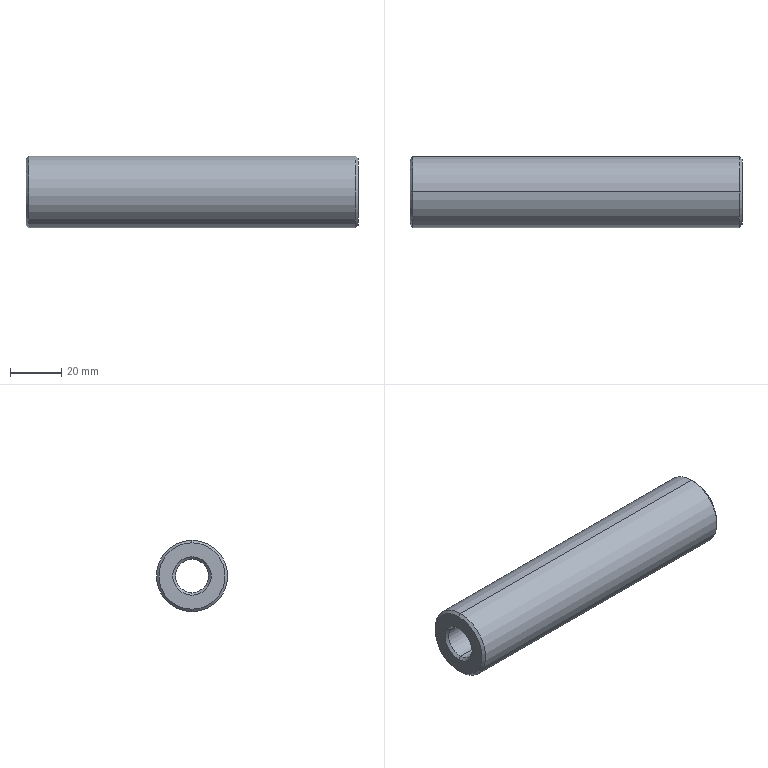Component | SolidWorks | LocatingGuideBushing130-2 | 1 solid | 14 faces | box 130 x 28 x 28 mm | volume 62664 mm3 | cone 8 | cylinder 4 | plane 2 | commonest cylinder face diameters 13 x2 28 x2
build123d program:
from build123d import *

# Parameters (mm, degrees)
SKETCH1_R           = 14
SKETCH1_R_2         = 6.5
BOSS_EXTRUDE1_DEPTH = 130
CHAMFER1_SIZE       = 1


with BuildPart() as part:
    # Sketch1 → Boss-Extrude1 (new body)
    with BuildSketch(Plane.XY):
        Circle(SKETCH1_R)
        Circle(SKETCH1_R_2, mode=Mode.SUBTRACT)
    extrude(amount=BOSS_EXTRUDE1_DEPTH)

    # Chamfer1
    chamfer1_edges = [part.edges().sort_by_distance(p)[0] for p in [
        (-14, 0, 0),
        (-14, 0, 130),
        (-6.5, 0, 0),
        (-6.5, 0, 130),
    ]]
    chamfer(chamfer1_edges, length=CHAMFER1_SIZE)


solid = part.part

# Placed as in the assembly
solid = solid.moved(Location((-197.809, 220.819, 0), (0, 90, 0)))
STEP:
#1=CARTESIAN_POINT('',(-2.67,8.694,-0.5118));
#2=VERTEX_POINT('',#1);
#3=CARTESIAN_POINT('',(-2.67,8.694,0.5118));
#4=VERTEX_POINT('',#3);
#5=CARTESIAN_POINT('',(-2.67,8.694,0.));
#6=DIRECTION('',(1.,-0.,0.));
#7=DIRECTION('',(0.,0.,-1.));
#8=AXIS2_PLACEMENT_3D('',#5,#6,#7);
#9=CIRCLE('',#8,0.5118);
#10=EDGE_CURVE('',#2,#4,#9,.T.);
#11=ORIENTED_EDGE('',*,*,#10,.F.);
#12=CARTESIAN_POINT('',(-2.709,8.694,-0.5512));
#13=VERTEX_POINT('',#12);
#14=CARTESIAN_POINT('',(-2.67,8.694,-0.5118));
#15=DIRECTION('',(-0.7071,0.,-0.7071));
#16=VECTOR('',#15,39.37);
#17=LINE('',#14,#16);
#18=EDGE_CURVE('',#2,#13,#17,.T.);
#19=ORIENTED_EDGE('',*,*,#18,.T.);
#20=CARTESIAN_POINT('',(-2.709,8.694,0.5512));
#21=VERTEX_POINT('',#20);
#22=CARTESIAN_POINT('',(-2.709,8.694,0.));
#23=DIRECTION('',(-1.,0.,-0.));
#24=DIRECTION('',(0.,-0.,-1.));
#25=AXIS2_PLACEMENT_3D('',#22,#23,#24);
#26=CIRCLE('',#25,0.5512);
#27=EDGE_CURVE('',#21,#13,#26,.T.);
#28=ORIENTED_EDGE('',*,*,#27,.F.);
#29=CARTESIAN_POINT('',(-2.67,8.694,0.5118));
#30=DIRECTION('',(-0.7071,-0.,0.7071));
#31=VECTOR('',#30,39.37);
#32=LINE('',#29,#31);
#33=EDGE_CURVE('',#4,#21,#32,.T.);
#34=ORIENTED_EDGE('',*,*,#33,.F.);
#35=EDGE_LOOP('',(#11,#19,#28,#34));
#36=FACE_OUTER_BOUND('',#35,.T.);
#37=CARTESIAN_POINT('',(-2.67,8.694,0.));
#38=DIRECTION('',(-1.,0.,-0.));
#39=DIRECTION('',(0.,0.,1.));
#40=AXIS2_PLACEMENT_3D('',#37,#38,#39);
#41=CONICAL_SURFACE('',#40,0.5118,0.7854);
#42=ADVANCED_FACE('',(#36),#41,.T.);
#43=CARTESIAN_POINT('',(-2.709,8.694,0.2559));
#44=VERTEX_POINT('',#43);
#45=CARTESIAN_POINT('',(-2.709,8.694,-0.2559));
#46=VERTEX_POINT('',#45);
#47=CARTESIAN_POINT('',(-2.709,8.694,0.));
#48=DIRECTION('',(1.,-0.,0.));
#49=DIRECTION('',(0.,0.,-1.));
#50=AXIS2_PLACEMENT_3D('',#47,#48,#49);
#51=CIRCLE('',#50,0.2559);
#52=EDGE_CURVE('',#44,#46,#51,.T.);
#53=ORIENTED_EDGE('',*,*,#52,.F.);
#54=CARTESIAN_POINT('',(-2.67,8.694,0.2953));
#55=VERTEX_POINT('',#54);
#56=CARTESIAN_POINT('',(-2.709,8.694,0.2559));
#57=DIRECTION('',(0.7071,-0.,0.7071));
#58=VECTOR('',#57,39.37);
#59=LINE('',#56,#58);
#60=EDGE_CURVE('',#44,#55,#59,.T.);
#61=ORIENTED_EDGE('',*,*,#60,.T.);
#62=CARTESIAN_POINT('',(-2.67,8.694,-0.2953));
#63=VERTEX_POINT('',#62);
#64=CARTESIAN_POINT('',(-2.67,8.694,0.));
#65=DIRECTION('',(-1.,0.,-0.));
#66=DIRECTION('',(0.,0.,-1.));
#67=AXIS2_PLACEMENT_3D('',#64,#65,#66);
#68=CIRCLE('',#67,0.2953);
#69=EDGE_CURVE('',#63,#55,#68,.T.);
#70=ORIENTED_EDGE('',*,*,#69,.F.);
#71=CARTESIAN_POINT('',(-2.709,8.694,-0.2559));
#72=DIRECTION('',(0.7071,0.,-0.7071));
#73=VECTOR('',#72,39.37);
#74=LINE('',#71,#73);
#75=EDGE_CURVE('',#46,#63,#74,.T.);
#76=ORIENTED_EDGE('',*,*,#75,.F.);
#77=EDGE_LOOP('',(#53,#61,#70,#76));
#78=FACE_OUTER_BOUND('',#77,.T.);
#79=CARTESIAN_POINT('',(-2.709,8.694,0.));
#80=DIRECTION('',(1.,-0.,0.));
#81=DIRECTION('',(0.,0.,-1.));
#82=AXIS2_PLACEMENT_3D('',#79,#80,#81);
#83=CONICAL_SURFACE('',#82,0.2559,0.7854);
#84=ADVANCED_FACE('',(#78),#83,.F.);
#85=CARTESIAN_POINT('',(-7.788,8.694,0.5118));
#86=VERTEX_POINT('',#85);
#87=CARTESIAN_POINT('',(-7.788,8.694,-0.5118));
#88=VERTEX_POINT('',#87);
#89=CARTESIAN_POINT('',(-7.788,8.694,0.));
#90=DIRECTION('',(-1.,0.,-0.));
#91=DIRECTION('',(0.,0.,-1.));
#92=AXIS2_PLACEMENT_3D('',#89,#90,#91);
#93=CIRCLE('',#92,0.5118);
#94=EDGE_CURVE('',#86,#88,#93,.T.);
#95=ORIENTED_EDGE('',*,*,#94,.F.);
#96=CARTESIAN_POINT('',(-7.748,8.694,0.5512));
#97=VERTEX_POINT('',#96);
#98=CARTESIAN_POINT('',(-7.748,8.694,0.5512));
#99=DIRECTION('',(0.7071,-0.,0.7071));
#100=VECTOR('',#99,39.37);
#101=LINE('',#98,#100);
#102=EDGE_CURVE('',#86,#97,#101,.T.);
#103=ORIENTED_EDGE('',*,*,#102,.T.);
#104=CARTESIAN_POINT('',(-7.748,8.694,-0.5512));
#105=VERTEX_POINT('',#104);
#106=CARTESIAN_POINT('',(-7.748,8.694,0.));
#107=DIRECTION('',(1.,-0.,0.));
#108=DIRECTION('',(0.,0.,-1.));
#109=AXIS2_PLACEMENT_3D('',#106,#107,#108);
#110=CIRCLE('',#109,0.5512);
#111=EDGE_CURVE('',#105,#97,#110,.T.);
#112=ORIENTED_EDGE('',*,*,#111,.F.);
#113=CARTESIAN_POINT('',(-7.748,8.694,-0.5512));
#114=DIRECTION('',(0.7071,0.,-0.7071));
#115=VECTOR('',#114,39.37);
#116=LINE('',#113,#115);
#117=EDGE_CURVE('',#88,#105,#116,.T.);
#118=ORIENTED_EDGE('',*,*,#117,.F.);
#119=EDGE_LOOP('',(#95,#103,#112,#118));
#120=FACE_OUTER_BOUND('',#119,.T.);
#121=CARTESIAN_POINT('',(-7.748,8.694,0.));
#122=DIRECTION('',(1.,-0.,0.));
#123=DIRECTION('',(0.,0.,-1.));
#124=AXIS2_PLACEMENT_3D('',#121,#122,#123);
#125=CONICAL_SURFACE('',#124,0.5512,0.7854);
#126=ADVANCED_FACE('',(#120),#125,.T.);
#127=CARTESIAN_POINT('',(-7.748,8.694,-0.2559));
#128=VERTEX_POINT('',#127);
#129=CARTESIAN_POINT('',(-7.748,8.694,0.2559));
#130=VERTEX_POINT('',#129);
#131=CARTESIAN_POINT('',(-7.748,8.694,0.));
#132=DIRECTION('',(-1.,0.,-0.));
#133=DIRECTION('',(0.,0.,-1.));
#134=AXIS2_PLACEMENT_3D('',#131,#132,#133);
#135=CIRCLE('',#134,0.2559);
#136=EDGE_CURVE('',#128,#130,#135,.T.);
#137=ORIENTED_EDGE('',*,*,#136,.F.);
#138=CARTESIAN_POINT('',(-7.788,8.694,-0.2953));
#139=VERTEX_POINT('',#138);
#140=CARTESIAN_POINT('',(-7.788,8.694,-0.2953));
#141=DIRECTION('',(-0.7071,0.,-0.7071));
#142=VECTOR('',#141,39.37);
#143=LINE('',#140,#142);
#144=EDGE_CURVE('',#128,#139,#143,.T.);
#145=ORIENTED_EDGE('',*,*,#144,.T.);
#146=CARTESIAN_POINT('',(-7.788,8.694,0.2953));
#147=VERTEX_POINT('',#146);
#148=CARTESIAN_POINT('',(-7.788,8.694,0.));
#149=DIRECTION('',(1.,-0.,0.));
#150=DIRECTION('',(0.,0.,-1.));
#151=AXIS2_PLACEMENT_3D('',#148,#149,#150);
#152=CIRCLE('',#151,0.2953);
#153=EDGE_CURVE('',#147,#139,#152,.T.);
#154=ORIENTED_EDGE('',*,*,#153,.F.);
#155=CARTESIAN_POINT('',(-7.788,8.694,0.2953));
#156=DIRECTION('',(-0.7071,-0.,0.7071));
#157=VECTOR('',#156,39.37);
#158=LINE('',#155,#157);
#159=EDGE_CURVE('',#130,#147,#158,.T.);
#160=ORIENTED_EDGE('',*,*,#159,.F.);
#161=EDGE_LOOP('',(#137,#145,#154,#160));
#162=FACE_OUTER_BOUND('',#161,.T.);
#163=CARTESIAN_POINT('',(-7.788,8.694,0.));
#164=DIRECTION('',(-1.,0.,-0.));
#165=DIRECTION('',(0.,0.,1.));
#166=AXIS2_PLACEMENT_3D('',#163,#164,#165);
#167=CONICAL_SURFACE('',#166,0.2953,0.7854);
#168=ADVANCED_FACE('',(#162),#167,.F.);
#169=ORIENTED_EDGE('',*,*,#52,.T.);
#170=CARTESIAN_POINT('',(-2.67,8.694,-0.2559));
#171=DIRECTION('',(-1.,0.,-0.));
#172=VECTOR('',#171,39.37);
#173=LINE('',#170,#172);
#174=EDGE_CURVE('',#46,#128,#173,.T.);
#175=ORIENTED_EDGE('',*,*,#174,.T.);
#176=ORIENTED_EDGE('',*,*,#136,.T.);
#177=CARTESIAN_POINT('',(-2.67,8.694,0.2559));
#178=DIRECTION('',(-1.,0.,-0.));
#179=VECTOR('',#178,39.37);
#180=LINE('',#177,#179);
#181=EDGE_CURVE('',#44,#130,#180,.T.);
#182=ORIENTED_EDGE('',*,*,#181,.F.);
#183=EDGE_LOOP('',(#169,#175,#176,#182));
#184=FACE_OUTER_BOUND('',#183,.T.);
#185=CARTESIAN_POINT('',(-2.67,8.694,0.));
#186=DIRECTION('',(-1.,0.,-0.));
#187=DIRECTION('',(0.,0.,1.));
#188=AXIS2_PLACEMENT_3D('',#185,#186,#187);
#189=CYLINDRICAL_SURFACE('',#188,0.2559);
#190=ADVANCED_FACE('',(#184),#189,.F.);
#191=ORIENTED_EDGE('',*,*,#27,.T.);
#192=CARTESIAN_POINT('',(-2.67,8.694,-0.5512));
#193=DIRECTION('',(-1.,0.,-0.));
#194=VECTOR('',#193,39.37);
#195=LINE('',#192,#194);
#196=EDGE_CURVE('',#13,#105,#195,.T.);
#197=ORIENTED_EDGE('',*,*,#196,.T.);
#198=ORIENTED_EDGE('',*,*,#111,.T.);
#199=CARTESIAN_POINT('',(-2.67,8.694,0.5512));
#200=DIRECTION('',(-1.,0.,-0.));
#201=VECTOR('',#200,39.37);
#202=LINE('',#199,#201);
#203=EDGE_CURVE('',#21,#97,#202,.T.);
#204=ORIENTED_EDGE('',*,*,#203,.F.);
#205=EDGE_LOOP('',(#191,#197,#198,#204));
#206=FACE_OUTER_BOUND('',#205,.T.);
#207=CARTESIAN_POINT('',(-2.67,8.694,0.));
#208=DIRECTION('',(-1.,0.,-0.));
#209=DIRECTION('',(0.,0.,1.));
#210=AXIS2_PLACEMENT_3D('',#207,#208,#209);
#211=CYLINDRICAL_SURFACE('',#210,0.5512);
#212=ADVANCED_FACE('',(#206),#211,.T.);
#213=ORIENTED_EDGE('',*,*,#69,.T.);
#214=CARTESIAN_POINT('',(-2.67,8.694,0.));
#215=DIRECTION('',(-1.,0.,-0.));
#216=DIRECTION('',(0.,0.,-1.));
#217=AXIS2_PLACEMENT_3D('',#214,#215,#216);
#218=CIRCLE('',#217,0.2953);
#219=EDGE_CURVE('',#55,#63,#218,.T.);
#220=ORIENTED_EDGE('',*,*,#219,.T.);
#221=EDGE_LOOP('',(#213,#220));
#222=FACE_BOUND('',#221,.T.);
#223=CARTESIAN_POINT('',(-2.67,8.694,0.));
#224=DIRECTION('',(1.,-0.,0.));
#225=DIRECTION('',(0.,0.,-1.));
#226=AXIS2_PLACEMENT_3D('',#223,#224,#225);
#227=CIRCLE('',#226,0.5118);
#228=EDGE_CURVE('',#4,#2,#227,.T.);
#229=ORIENTED_EDGE('',*,*,#228,.T.);
#230=ORIENTED_EDGE('',*,*,#10,.T.);
#231=EDGE_LOOP('',(#229,#230));
#232=FACE_OUTER_BOUND('',#231,.T.);
#233=CARTESIAN_POINT('',(-2.67,8.694,0.));
#234=DIRECTION('',(1.,-0.,0.));
#235=DIRECTION('',(0.,0.,-1.));
#236=AXIS2_PLACEMENT_3D('',#233,#234,#235);
#237=PLANE('',#236);
#238=ADVANCED_FACE('',(#222,#232),#237,.T.);
#239=ORIENTED_EDGE('',*,*,#153,.T.);
#240=CARTESIAN_POINT('',(-7.788,8.694,0.));
#241=DIRECTION('',(1.,-0.,0.));
#242=DIRECTION('',(0.,0.,-1.));
#243=AXIS2_PLACEMENT_3D('',#240,#241,#242);
#244=CIRCLE('',#243,0.2953);
#245=EDGE_CURVE('',#139,#147,#244,.T.);
#246=ORIENTED_EDGE('',*,*,#245,.T.);
#247=EDGE_LOOP('',(#239,#246));
#248=FACE_BOUND('',#247,.T.);
#249=CARTESIAN_POINT('',(-7.788,8.694,0.));
#250=DIRECTION('',(-1.,0.,-0.));
#251=DIRECTION('',(0.,0.,-1.));
#252=AXIS2_PLACEMENT_3D('',#249,#250,#251);
#253=CIRCLE('',#252,0.5118);
#254=EDGE_CURVE('',#88,#86,#253,.T.);
#255=ORIENTED_EDGE('',*,*,#254,.T.);
#256=ORIENTED_EDGE('',*,*,#94,.T.);
#257=EDGE_LOOP('',(#255,#256));
#258=FACE_OUTER_BOUND('',#257,.T.);
#259=CARTESIAN_POINT('',(-7.788,8.694,0.));
#260=DIRECTION('',(1.,-0.,0.));
#261=DIRECTION('',(0.,0.,-1.));
#262=AXIS2_PLACEMENT_3D('',#259,#260,#261);
#263=PLANE('',#262);
#264=ADVANCED_FACE('',(#248,#258),#263,.F.);
#265=ORIENTED_EDGE('',*,*,#196,.F.);
#266=CARTESIAN_POINT('',(-2.709,8.694,0.));
#267=DIRECTION('',(-1.,0.,-0.));
#268=DIRECTION('',(0.,0.,-1.));
#269=AXIS2_PLACEMENT_3D('',#266,#267,#268);
#270=CIRCLE('',#269,0.5512);
#271=EDGE_CURVE('',#13,#21,#270,.T.);
#272=ORIENTED_EDGE('',*,*,#271,.T.);
#273=ORIENTED_EDGE('',*,*,#203,.T.);
#274=CARTESIAN_POINT('',(-7.748,8.694,0.));
#275=DIRECTION('',(1.,-0.,0.));
#276=DIRECTION('',(0.,0.,-1.));
#277=AXIS2_PLACEMENT_3D('',#274,#275,#276);
#278=CIRCLE('',#277,0.5512);
#279=EDGE_CURVE('',#97,#105,#278,.T.);
#280=ORIENTED_EDGE('',*,*,#279,.T.);
#281=EDGE_LOOP('',(#265,#272,#273,#280));
#282=FACE_OUTER_BOUND('',#281,.T.);
#283=CARTESIAN_POINT('',(-2.67,8.694,0.));
#284=DIRECTION('',(-1.,0.,-0.));
#285=DIRECTION('',(0.,0.,1.));
#286=AXIS2_PLACEMENT_3D('',#283,#284,#285);
#287=CYLINDRICAL_SURFACE('',#286,0.5512);
#288=ADVANCED_FACE('',(#282),#287,.T.);
#289=ORIENTED_EDGE('',*,*,#174,.F.);
#290=CARTESIAN_POINT('',(-2.709,8.694,0.));
#291=DIRECTION('',(1.,-0.,0.));
#292=DIRECTION('',(0.,0.,-1.));
#293=AXIS2_PLACEMENT_3D('',#290,#291,#292);
#294=CIRCLE('',#293,0.2559);
#295=EDGE_CURVE('',#46,#44,#294,.T.);
#296=ORIENTED_EDGE('',*,*,#295,.T.);
#297=ORIENTED_EDGE('',*,*,#181,.T.);
#298=CARTESIAN_POINT('',(-7.748,8.694,0.));
#299=DIRECTION('',(-1.,0.,-0.));
#300=DIRECTION('',(0.,0.,-1.));
#301=AXIS2_PLACEMENT_3D('',#298,#299,#300);
#302=CIRCLE('',#301,0.2559);
#303=EDGE_CURVE('',#130,#128,#302,.T.);
#304=ORIENTED_EDGE('',*,*,#303,.T.);
#305=EDGE_LOOP('',(#289,#296,#297,#304));
#306=FACE_OUTER_BOUND('',#305,.T.);
#307=CARTESIAN_POINT('',(-2.67,8.694,0.));
#308=DIRECTION('',(-1.,0.,-0.));
#309=DIRECTION('',(0.,0.,1.));
#310=AXIS2_PLACEMENT_3D('',#307,#308,#309);
#311=CYLINDRICAL_SURFACE('',#310,0.2559);
#312=ADVANCED_FACE('',(#306),#311,.F.);
#313=ORIENTED_EDGE('',*,*,#144,.F.);
#314=ORIENTED_EDGE('',*,*,#303,.F.);
#315=ORIENTED_EDGE('',*,*,#159,.T.);
#316=ORIENTED_EDGE('',*,*,#245,.F.);
#317=EDGE_LOOP('',(#313,#314,#315,#316));
#318=FACE_OUTER_BOUND('',#317,.T.);
#319=CARTESIAN_POINT('',(-7.788,8.694,0.));
#320=DIRECTION('',(-1.,0.,-0.));
#321=DIRECTION('',(0.,0.,1.));
#322=AXIS2_PLACEMENT_3D('',#319,#320,#321);
#323=CONICAL_SURFACE('',#322,0.2953,0.7854);
#324=ADVANCED_FACE('',(#318),#323,.F.);
#325=ORIENTED_EDGE('',*,*,#102,.F.);
#326=ORIENTED_EDGE('',*,*,#254,.F.);
#327=ORIENTED_EDGE('',*,*,#117,.T.);
#328=ORIENTED_EDGE('',*,*,#279,.F.);
#329=EDGE_LOOP('',(#325,#326,#327,#328));
#330=FACE_OUTER_BOUND('',#329,.T.);
#331=CARTESIAN_POINT('',(-7.748,8.694,0.));
#332=DIRECTION('',(1.,-0.,0.));
#333=DIRECTION('',(0.,0.,-1.));
#334=AXIS2_PLACEMENT_3D('',#331,#332,#333);
#335=CONICAL_SURFACE('',#334,0.5512,0.7854);
#336=ADVANCED_FACE('',(#330),#335,.T.);
#337=ORIENTED_EDGE('',*,*,#60,.F.);
#338=ORIENTED_EDGE('',*,*,#295,.F.);
#339=ORIENTED_EDGE('',*,*,#75,.T.);
#340=ORIENTED_EDGE('',*,*,#219,.F.);
#341=EDGE_LOOP('',(#337,#338,#339,#340));
#342=FACE_OUTER_BOUND('',#341,.T.);
#343=CARTESIAN_POINT('',(-2.709,8.694,0.));
#344=DIRECTION('',(1.,-0.,0.));
#345=DIRECTION('',(0.,0.,-1.));
#346=AXIS2_PLACEMENT_3D('',#343,#344,#345);
#347=CONICAL_SURFACE('',#346,0.2559,0.7854);
#348=ADVANCED_FACE('',(#342),#347,.F.);
#349=ORIENTED_EDGE('',*,*,#18,.F.);
#350=ORIENTED_EDGE('',*,*,#228,.F.);
#351=ORIENTED_EDGE('',*,*,#33,.T.);
#352=ORIENTED_EDGE('',*,*,#271,.F.);
#353=EDGE_LOOP('',(#349,#350,#351,#352));
#354=FACE_OUTER_BOUND('',#353,.T.);
#355=CARTESIAN_POINT('',(-2.67,8.694,0.));
#356=DIRECTION('',(-1.,0.,-0.));
#357=DIRECTION('',(0.,0.,1.));
#358=AXIS2_PLACEMENT_3D('',#355,#356,#357);
#359=CONICAL_SURFACE('',#358,0.5118,0.7854);
#360=ADVANCED_FACE('',(#354),#359,.T.);
#361=CLOSED_SHELL('',(#42,#84,#126,#168,#190,#212,#238,#264,#288,#312,#324,#336,#348,#360));
#362=MANIFOLD_SOLID_BREP('',#361);
#363=CARTESIAN_POINT('',(0.,0.,0.));
#364=DIRECTION('',(0.,0.,1.));
#365=DIRECTION('',(1.,0.,0.));
#366=AXIS2_PLACEMENT_3D('',#363,#364,#365);
#367=(LENGTH_UNIT()NAMED_UNIT(*)SI_UNIT($,.METRE.));
#368=LENGTH_MEASURE_WITH_UNIT(LENGTH_MEASURE(0.0254),#367);
#369=DIMENSIONAL_EXPONENTS(1.,0.,0.,0.,0.,0.,0.);
#370=(CONVERSION_BASED_UNIT('',#368)LENGTH_UNIT()NAMED_UNIT(#369));
#371=UNCERTAINTY_MEASURE_WITH_UNIT(LENGTH_MEASURE(0.00001),#370,'','');
#372=(NAMED_UNIT(*)PLANE_ANGLE_UNIT()SI_UNIT($,.RADIAN.));
#373=(NAMED_UNIT(*)SI_UNIT($,.STERADIAN.)SOLID_ANGLE_UNIT());
#374=(GEOMETRIC_REPRESENTATION_CONTEXT(3)GLOBAL_UNCERTAINTY_ASSIGNED_CONTEXT((#371))GLOBAL_UNIT_ASSIGNED_CONTEXT((#370,#372,#373))REPRESENTATION_CONTEXT('',''));
#375=ADVANCED_BREP_SHAPE_REPRESENTATION('',(#362,#366),#374);
#376=COLOUR_RGB('',0.7922,0.8196,0.9333);
#377=FILL_AREA_STYLE_COLOUR('',#376);
#378=FILL_AREA_STYLE('',(#377));
#379=SURFACE_STYLE_FILL_AREA(#378);
#380=SURFACE_SIDE_STYLE('',(#379));
#381=SURFACE_STYLE_USAGE(.BOTH.,#380);
#382=PRESENTATION_STYLE_ASSIGNMENT((#381));
#383=STYLED_ITEM('',(#382),#362);
#384=(LENGTH_UNIT()NAMED_UNIT(*)SI_UNIT($,.METRE.));
#385=LENGTH_MEASURE_WITH_UNIT(LENGTH_MEASURE(0.0254),#384);
#386=DIMENSIONAL_EXPONENTS(1.,0.,0.,0.,0.,0.,0.);
#387=(CONVERSION_BASED_UNIT('',#385)LENGTH_UNIT()NAMED_UNIT(#386));
#388=UNCERTAINTY_MEASURE_WITH_UNIT(LENGTH_MEASURE(0.00001),#387,'','');
#389=(NAMED_UNIT(*)PLANE_ANGLE_UNIT()SI_UNIT($,.RADIAN.));
#390=(NAMED_UNIT(*)SI_UNIT($,.STERADIAN.)SOLID_ANGLE_UNIT());
#391=(GEOMETRIC_REPRESENTATION_CONTEXT(3)GLOBAL_UNCERTAINTY_ASSIGNED_CONTEXT((#388))GLOBAL_UNIT_ASSIGNED_CONTEXT((#387,#389,#390))REPRESENTATION_CONTEXT('',''));
#392=MECHANICAL_DESIGN_GEOMETRIC_PRESENTATION_REPRESENTATION('',(#383),#391);
#393=PRESENTATION_LAYER_ASSIGNMENT('','',(#383));